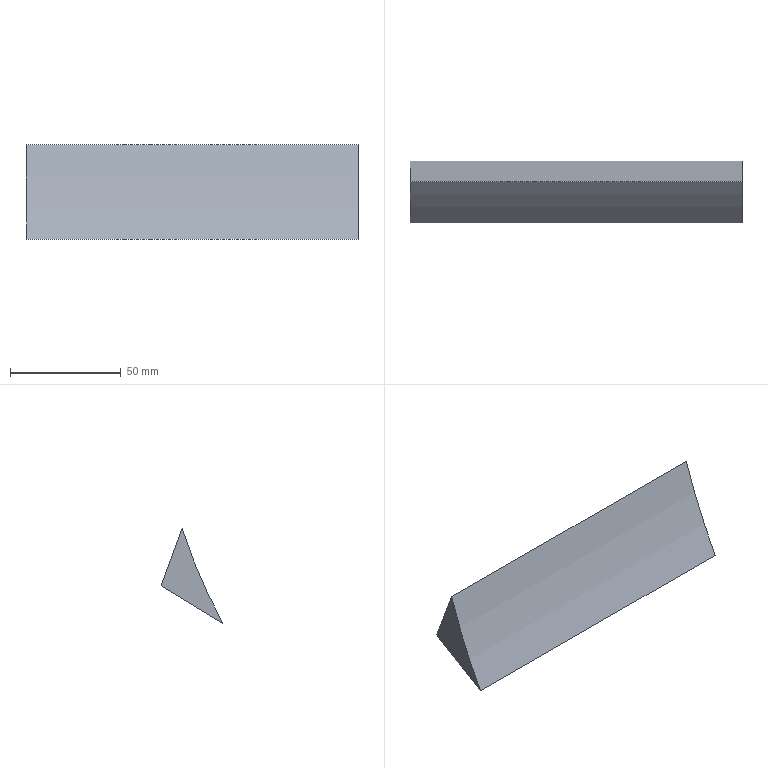Component | SolidWorks | SAV1-3 | 1 solid | 5 faces | box 150 x 27.92 x 42.85 mm | volume 61411 mm3 | plane 4 | cylinder 1 | commonest cylinder face diameters 521 x1
build123d program:
from build123d import *

# Parameters (mm, degrees)
BOSS_EXTRUDE1_DEPTH = 150


with BuildPart() as part:
    # Sketch1 → Boss-Extrude1 (new body)
    with BuildSketch(Plane.XY):
        with BuildLine():
            Line((0, 25), (23.089, 1.911))
            ThreePointArc((23.089, 1.911), (0.2583, 6.805), (-22.919, 9.635))
            Line((-22.919, 9.635), (0, 25))
        make_face()
    extrude(amount=-BOSS_EXTRUDE1_DEPTH)


solid = part.part

# Placed as in the assembly
solid = solid.moved(Location((-710, 232.733, -101.11), (-13.755, 90, 0)))
STEP:
#1=CARTESIAN_POINT('',(-33.858,9.746,-3.194));
#2=VERTEX_POINT('',#1);
#3=CARTESIAN_POINT('',(-33.858,10.119,-4.215));
#4=VERTEX_POINT('',#3);
#5=CARTESIAN_POINT('',(-33.858,10.119,-4.215));
#6=DIRECTION('',(-0.,0.3434,-0.9392));
#7=VECTOR('',#6,39.37);
#8=LINE('',#5,#7);
#9=EDGE_CURVE('',#2,#4,#8,.T.);
#10=ORIENTED_EDGE('',*,*,#9,.F.);
#11=CARTESIAN_POINT('',(-27.953,9.746,-3.194));
#12=VERTEX_POINT('',#11);
#13=CARTESIAN_POINT('',(-35.885,9.746,-3.194));
#14=DIRECTION('',(1.,0.,0.));
#15=VECTOR('',#14,39.37);
#16=LINE('',#13,#15);
#17=EDGE_CURVE('',#2,#12,#16,.T.);
#18=ORIENTED_EDGE('',*,*,#17,.T.);
#19=CARTESIAN_POINT('',(-27.953,10.119,-4.215));
#20=VERTEX_POINT('',#19);
#21=CARTESIAN_POINT('',(-27.953,10.119,-4.215));
#22=DIRECTION('',(0.,-0.3434,0.9392));
#23=VECTOR('',#22,39.37);
#24=LINE('',#21,#23);
#25=EDGE_CURVE('',#20,#12,#24,.T.);
#26=ORIENTED_EDGE('',*,*,#25,.F.);
#27=CARTESIAN_POINT('',(-35.885,10.119,-4.215));
#28=DIRECTION('',(1.,0.,0.));
#29=VECTOR('',#28,39.37);
#30=LINE('',#27,#29);
#31=EDGE_CURVE('',#4,#20,#30,.T.);
#32=ORIENTED_EDGE('',*,*,#31,.F.);
#33=EDGE_LOOP('',(#10,#18,#26,#32));
#34=FACE_OUTER_BOUND('',#33,.T.);
#35=CARTESIAN_POINT('',(-35.885,10.119,-4.215));
#36=DIRECTION('',(-0.,0.9392,0.3434));
#37=DIRECTION('',(0.,-0.3434,0.9392));
#38=AXIS2_PLACEMENT_3D('',#35,#36,#37);
#39=PLANE('',#38);
#40=ADVANCED_FACE('',(#34),#39,.T.);
#41=CARTESIAN_POINT('',(-33.858,9.02,-4.882));
#42=VERTEX_POINT('',#41);
#43=CARTESIAN_POINT('',(-33.858,10.119,-4.215));
#44=DIRECTION('',(0.,-0.855,-0.5187));
#45=VECTOR('',#44,39.37);
#46=LINE('',#43,#45);
#47=EDGE_CURVE('',#4,#42,#46,.T.);
#48=ORIENTED_EDGE('',*,*,#47,.F.);
#49=ORIENTED_EDGE('',*,*,#31,.T.);
#50=CARTESIAN_POINT('',(-27.953,9.02,-4.882));
#51=VERTEX_POINT('',#50);
#52=CARTESIAN_POINT('',(-27.953,10.119,-4.215));
#53=DIRECTION('',(-0.,0.855,0.5187));
#54=VECTOR('',#53,39.37);
#55=LINE('',#52,#54);
#56=EDGE_CURVE('',#51,#20,#55,.T.);
#57=ORIENTED_EDGE('',*,*,#56,.F.);
#58=CARTESIAN_POINT('',(-35.885,9.02,-4.882));
#59=DIRECTION('',(1.,0.,0.));
#60=VECTOR('',#59,39.37);
#61=LINE('',#58,#60);
#62=EDGE_CURVE('',#42,#51,#61,.T.);
#63=ORIENTED_EDGE('',*,*,#62,.F.);
#64=EDGE_LOOP('',(#48,#49,#57,#63));
#65=FACE_OUTER_BOUND('',#64,.T.);
#66=CARTESIAN_POINT('',(-35.885,10.119,-4.215));
#67=DIRECTION('',(-0.,0.5187,-0.855));
#68=DIRECTION('',(-0.,0.855,0.5187));
#69=AXIS2_PLACEMENT_3D('',#66,#67,#68);
#70=PLANE('',#69);
#71=ADVANCED_FACE('',(#65),#70,.T.);
#72=CARTESIAN_POINT('',(-33.858,-0.,-0.));
#73=DIRECTION('',(1.,0.,-0.));
#74=DIRECTION('',(0.,-0.9713,0.2378));
#75=AXIS2_PLACEMENT_3D('',#72,#73,#74);
#76=CIRCLE('',#75,10.256);
#77=EDGE_CURVE('',#42,#2,#76,.T.);
#78=ORIENTED_EDGE('',*,*,#77,.F.);
#79=ORIENTED_EDGE('',*,*,#62,.T.);
#80=CARTESIAN_POINT('',(-27.953,-0.,-0.));
#81=DIRECTION('',(-1.,-0.,0.));
#82=DIRECTION('',(0.,-0.2378,-0.9713));
#83=AXIS2_PLACEMENT_3D('',#80,#81,#82);
#84=CIRCLE('',#83,10.256);
#85=EDGE_CURVE('',#12,#51,#84,.T.);
#86=ORIENTED_EDGE('',*,*,#85,.F.);
#87=ORIENTED_EDGE('',*,*,#17,.F.);
#88=EDGE_LOOP('',(#78,#79,#86,#87));
#89=FACE_OUTER_BOUND('',#88,.T.);
#90=CARTESIAN_POINT('',(-35.885,-0.,-0.));
#91=DIRECTION('',(1.,0.,0.));
#92=DIRECTION('',(0.,-0.2378,-0.9713));
#93=AXIS2_PLACEMENT_3D('',#90,#91,#92);
#94=CYLINDRICAL_SURFACE('',#93,10.256);
#95=ADVANCED_FACE('',(#89),#94,.F.);
#96=ORIENTED_EDGE('',*,*,#25,.T.);
#97=ORIENTED_EDGE('',*,*,#85,.T.);
#98=ORIENTED_EDGE('',*,*,#56,.T.);
#99=EDGE_LOOP('',(#96,#97,#98));
#100=FACE_OUTER_BOUND('',#99,.T.);
#101=CARTESIAN_POINT('',(-27.953,-0.,-0.));
#102=DIRECTION('',(1.,0.,-0.));
#103=DIRECTION('',(0.,-0.2378,-0.9713));
#104=AXIS2_PLACEMENT_3D('',#101,#102,#103);
#105=PLANE('',#104);
#106=ADVANCED_FACE('',(#100),#105,.T.);
#107=ORIENTED_EDGE('',*,*,#9,.T.);
#108=ORIENTED_EDGE('',*,*,#47,.T.);
#109=ORIENTED_EDGE('',*,*,#77,.T.);
#110=EDGE_LOOP('',(#107,#108,#109));
#111=FACE_OUTER_BOUND('',#110,.T.);
#112=CARTESIAN_POINT('',(-33.858,-0.,-0.));
#113=DIRECTION('',(1.,0.,-0.));
#114=DIRECTION('',(-0.,0.,-1.));
#115=AXIS2_PLACEMENT_3D('',#112,#113,#114);
#116=PLANE('',#115);
#117=ADVANCED_FACE('',(#111),#116,.F.);
#118=CLOSED_SHELL('',(#40,#71,#95,#106,#117));
#119=MANIFOLD_SOLID_BREP('',#118);
#120=CARTESIAN_POINT('',(0.,0.,0.));
#121=DIRECTION('',(0.,0.,1.));
#122=DIRECTION('',(1.,0.,0.));
#123=AXIS2_PLACEMENT_3D('',#120,#121,#122);
#124=(LENGTH_UNIT()NAMED_UNIT(*)SI_UNIT($,.METRE.));
#125=LENGTH_MEASURE_WITH_UNIT(LENGTH_MEASURE(0.0254),#124);
#126=DIMENSIONAL_EXPONENTS(1.,0.,0.,0.,0.,0.,0.);
#127=(CONVERSION_BASED_UNIT('',#125)LENGTH_UNIT()NAMED_UNIT(#126));
#128=UNCERTAINTY_MEASURE_WITH_UNIT(LENGTH_MEASURE(0.00001),#127,'','');
#129=(NAMED_UNIT(*)PLANE_ANGLE_UNIT()SI_UNIT($,.RADIAN.));
#130=(NAMED_UNIT(*)SI_UNIT($,.STERADIAN.)SOLID_ANGLE_UNIT());
#131=(GEOMETRIC_REPRESENTATION_CONTEXT(3)GLOBAL_UNCERTAINTY_ASSIGNED_CONTEXT((#128))GLOBAL_UNIT_ASSIGNED_CONTEXT((#127,#129,#130))REPRESENTATION_CONTEXT('',''));
#132=ADVANCED_BREP_SHAPE_REPRESENTATION('',(#119,#123),#131);
#133=COLOUR_RGB('',0.7922,0.8196,0.9333);
#134=FILL_AREA_STYLE_COLOUR('',#133);
#135=FILL_AREA_STYLE('',(#134));
#136=SURFACE_STYLE_FILL_AREA(#135);
#137=SURFACE_SIDE_STYLE('',(#136));
#138=SURFACE_STYLE_USAGE(.BOTH.,#137);
#139=PRESENTATION_STYLE_ASSIGNMENT((#138));
#140=STYLED_ITEM('',(#139),#119);
#141=PRESENTATION_LAYER_ASSIGNMENT('','',(#140));
#142=(LENGTH_UNIT()NAMED_UNIT(*)SI_UNIT($,.METRE.));
#143=LENGTH_MEASURE_WITH_UNIT(LENGTH_MEASURE(0.0254),#142);
#144=DIMENSIONAL_EXPONENTS(1.,0.,0.,0.,0.,0.,0.);
#145=(CONVERSION_BASED_UNIT('',#143)LENGTH_UNIT()NAMED_UNIT(#144));
#146=UNCERTAINTY_MEASURE_WITH_UNIT(LENGTH_MEASURE(0.00001),#145,'','');
#147=(NAMED_UNIT(*)PLANE_ANGLE_UNIT()SI_UNIT($,.RADIAN.));
#148=(NAMED_UNIT(*)SI_UNIT($,.STERADIAN.)SOLID_ANGLE_UNIT());
#149=(GEOMETRIC_REPRESENTATION_CONTEXT(3)GLOBAL_UNCERTAINTY_ASSIGNED_CONTEXT((#146))GLOBAL_UNIT_ASSIGNED_CONTEXT((#145,#147,#148))REPRESENTATION_CONTEXT('',''));
#150=MECHANICAL_DESIGN_GEOMETRIC_PRESENTATION_REPRESENTATION('',(#140),#149);